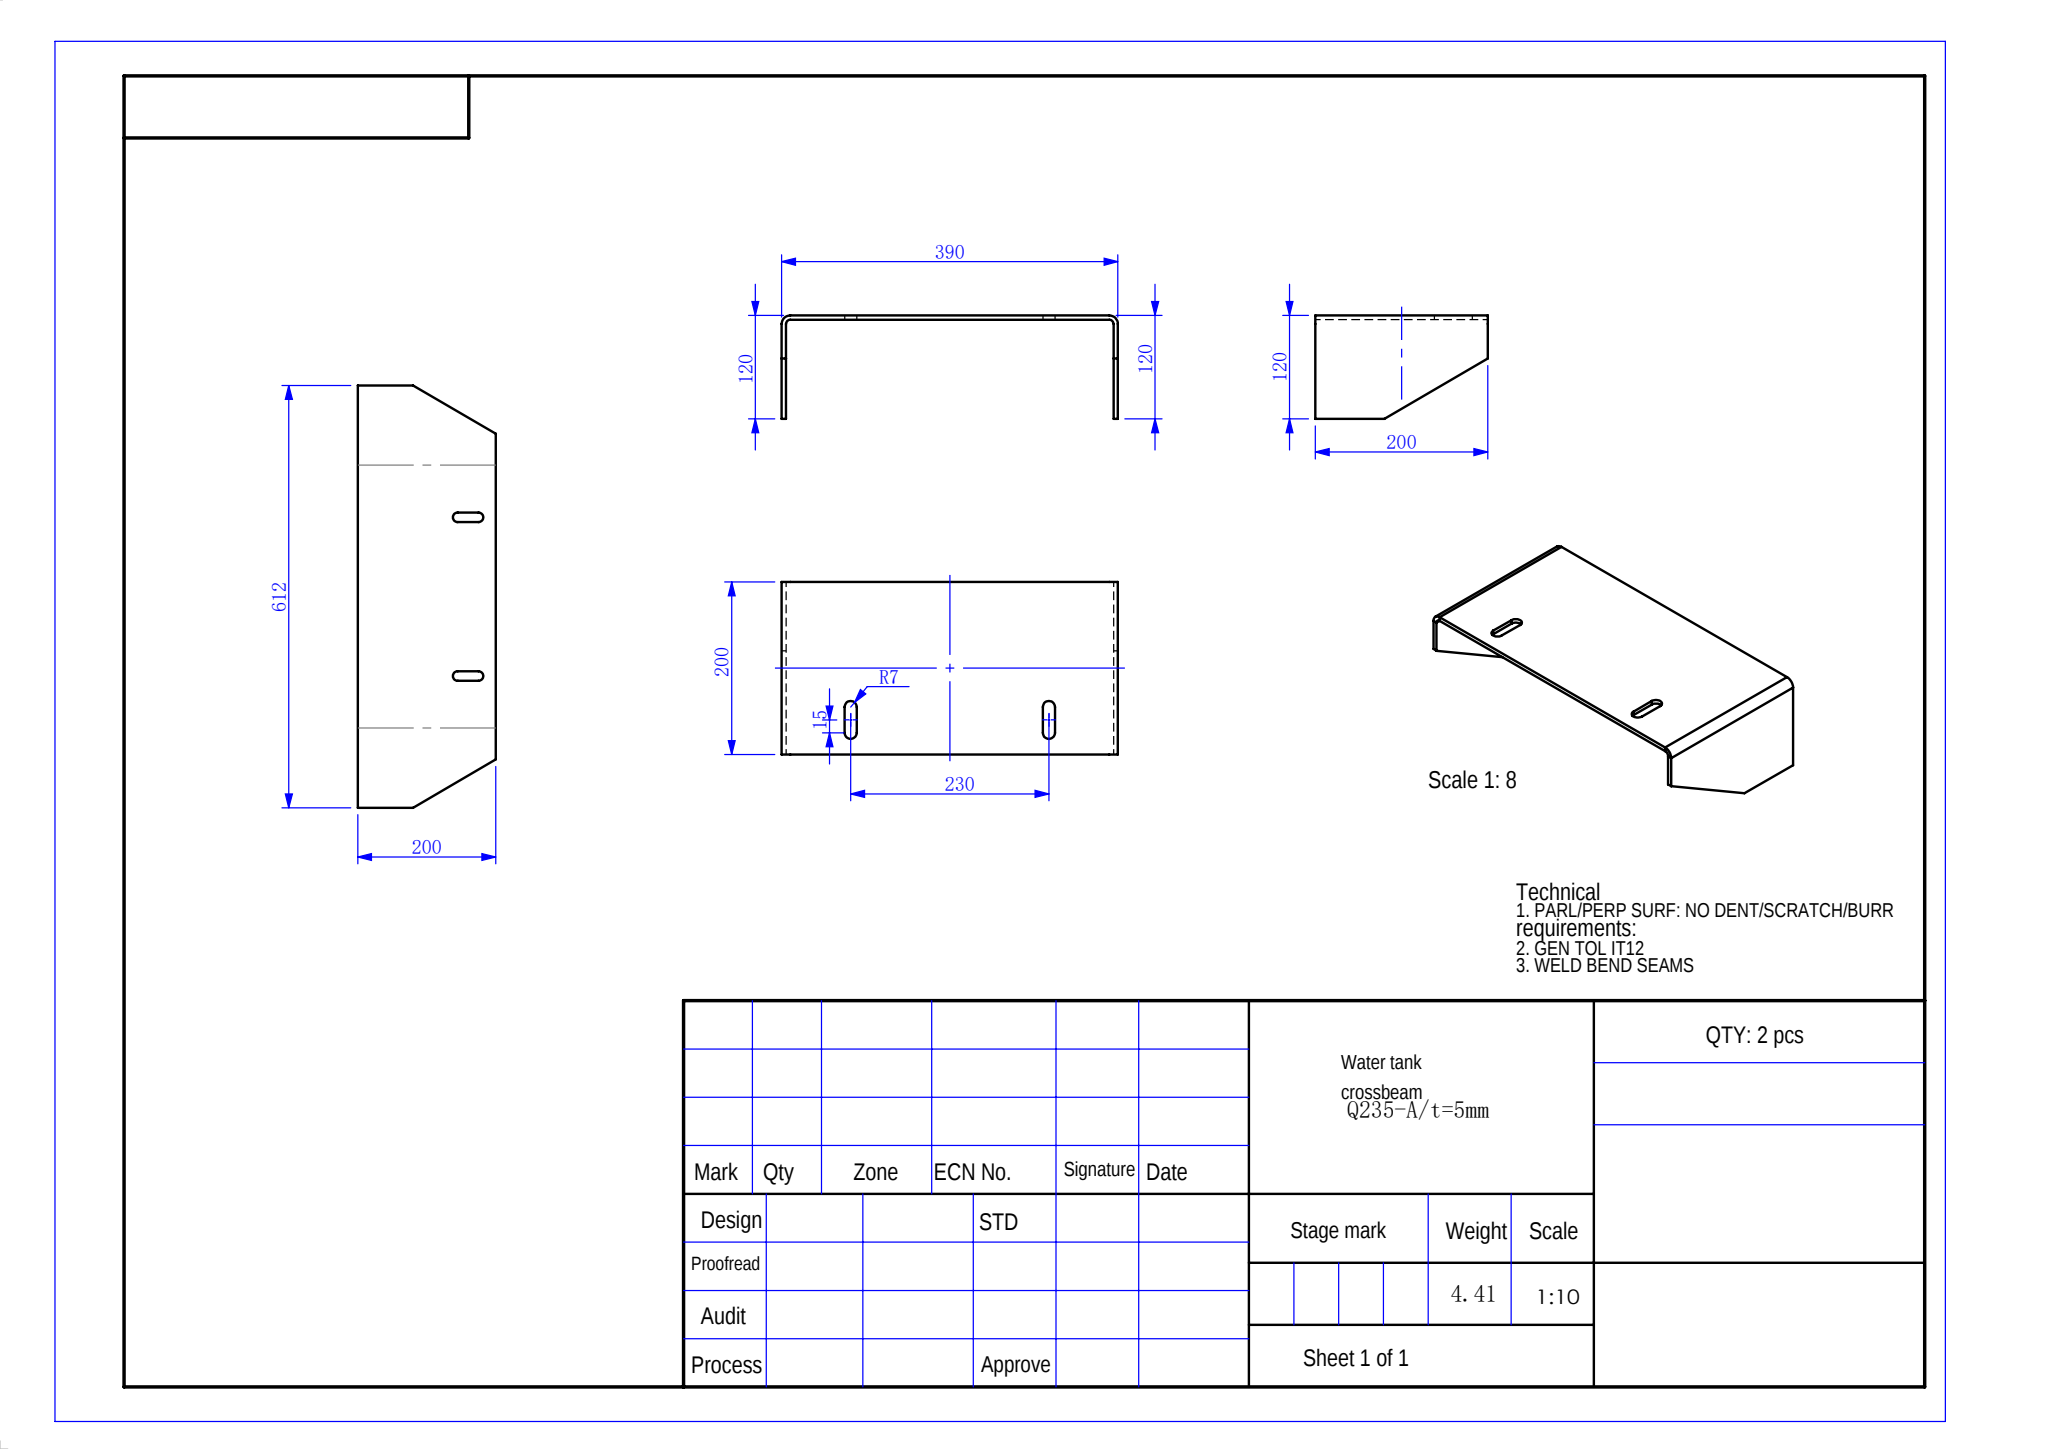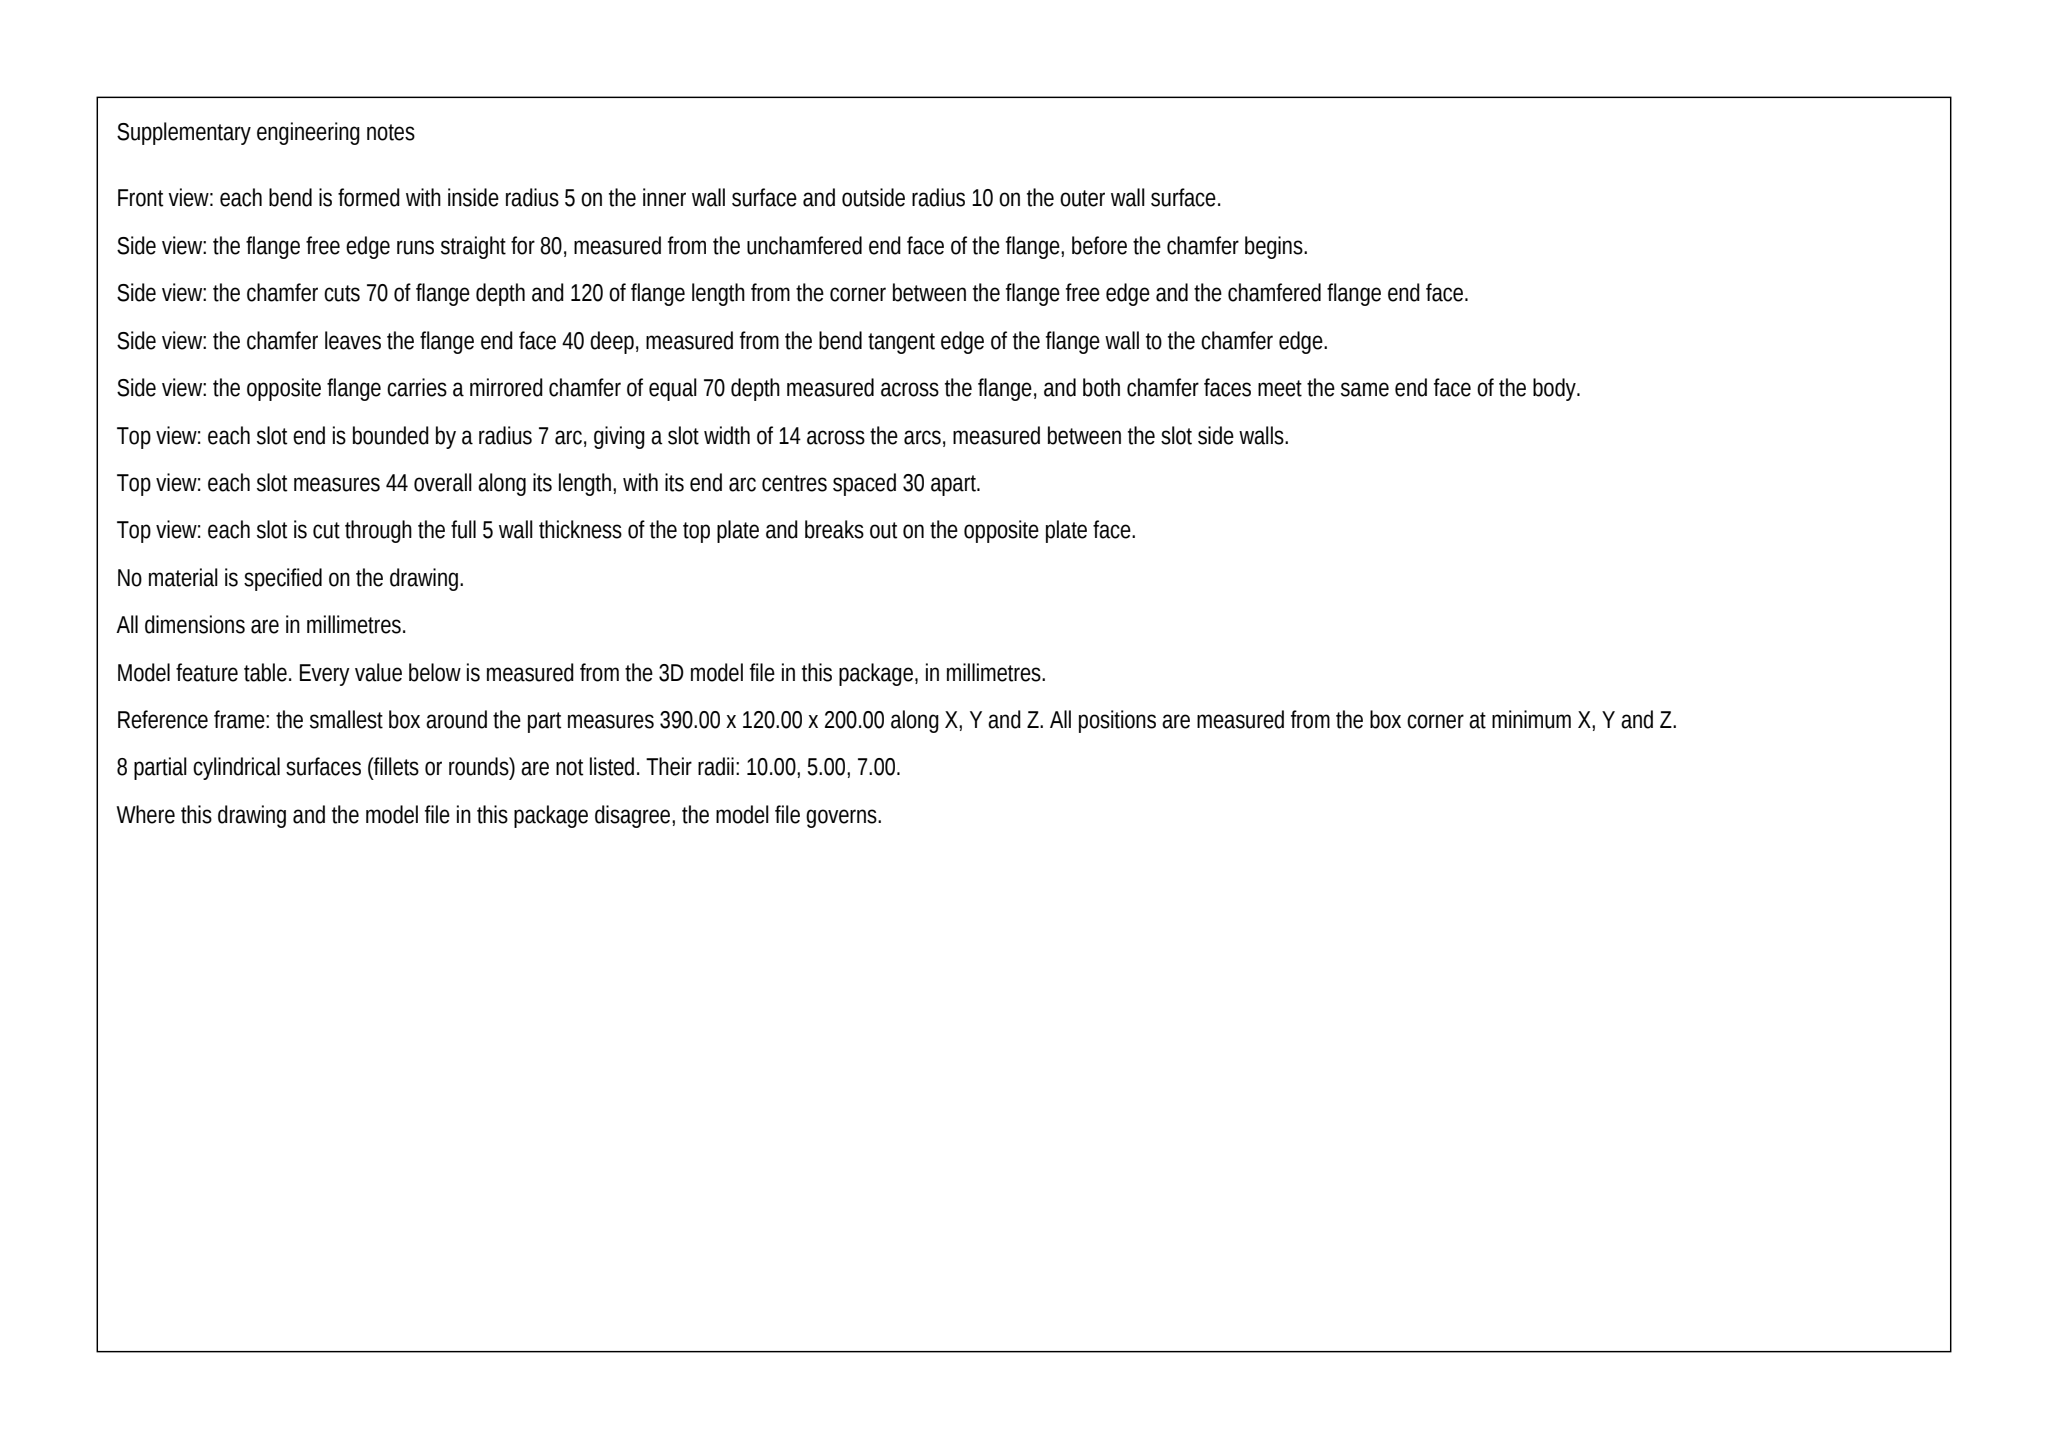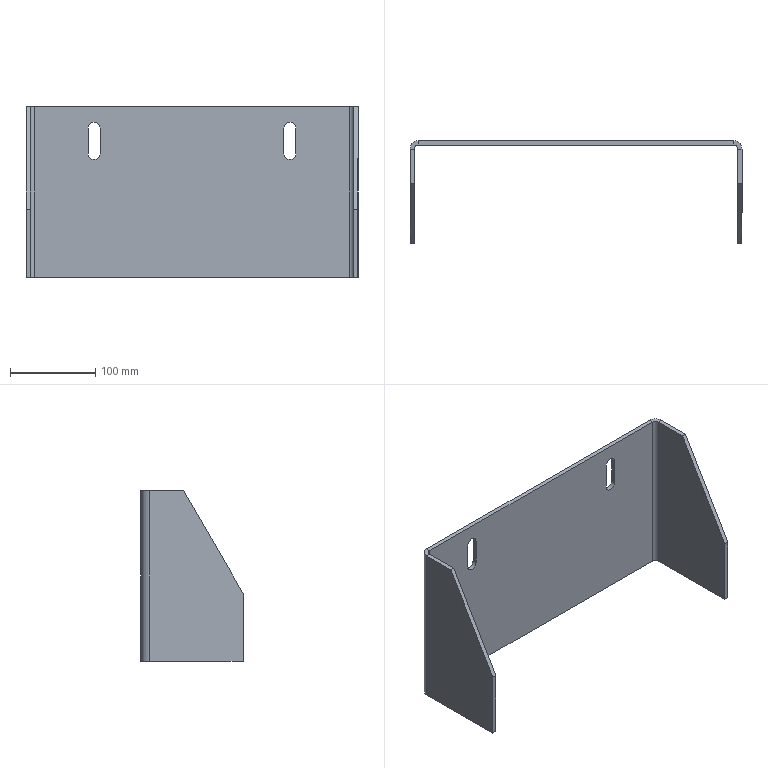Part | SolidWorks | mm | material Q235-A | 1 solid | 34 faces | box 390 x 120 x 200 mm | volume 565823 mm3 | plane 24 | cylinder 10 | commonest cylinder face diameters 14 x6 20 x2 10 x2
Drawing notes:
SLOT 14 WIDE x 30 LG, R7 ENDS, 16 BTWN END CTRS - 2 PL | from the solid: 4 x dia14 y-axis 180 deg arcs at z=145 & z=175 (pairs at x=80 and x=310); slot faces x=73/87 and x=303/317, z 145-175 -> 14 wide, 30 long, end ctrs 16 apart
SLOT CL 40 FROM NEAR 200 EDGE (SLOT 25 TO 55 FROM EDGE) | from the solid: slot z extent 145-175 of 200 depth -> 25 and 55 from z=200 edge, CL at 40
BEND R5 INSIDE, R10 OUTSIDE - TYP 2 PL (DELETE "44") | from the solid: concave dia10 z-arcs at (10,110) & (380,110); convex dia20 z-arcs same axes, 90 deg
SIDE VIEW: FLAT BOT EDGE 80 FROM END TO CHAMFER ("22"=80) | from the solid: y=0 faces x[0,5] & x[385,390], z 0-80; inclined plane starts at z=80
CHAMFER 70 x 120 ON SIDE LEG, 30.3 DEG - 2 PL ("33"=70) | from the solid: inclined planes bbox_from [0,0,80] & [385,0,80], size [5,70,120], angle 30.3 deg to Y
SLOT CL 40 FROM EDGE IN 200 DIR; 230 BTWN SLOT CLS | from the solid: slot CLs x=80 & x=310 -> 230 apart; slot CL z=160, i.e. 40 from z=200 edge